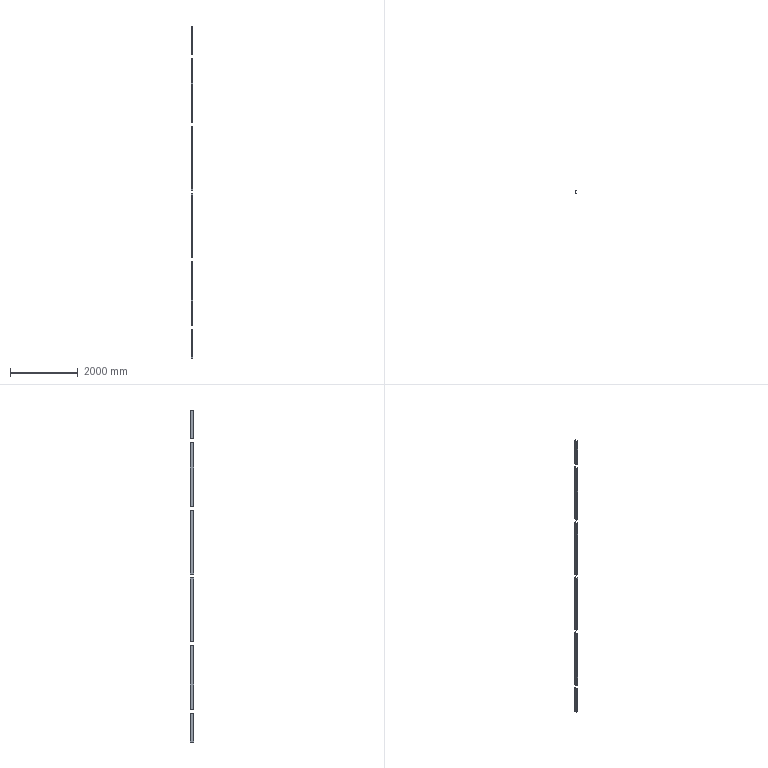Component | NX | CHUNSHUIJINCAO_CAOGANG | 6 solids | 60 faces | volume 11591957 mm3 | plane 60